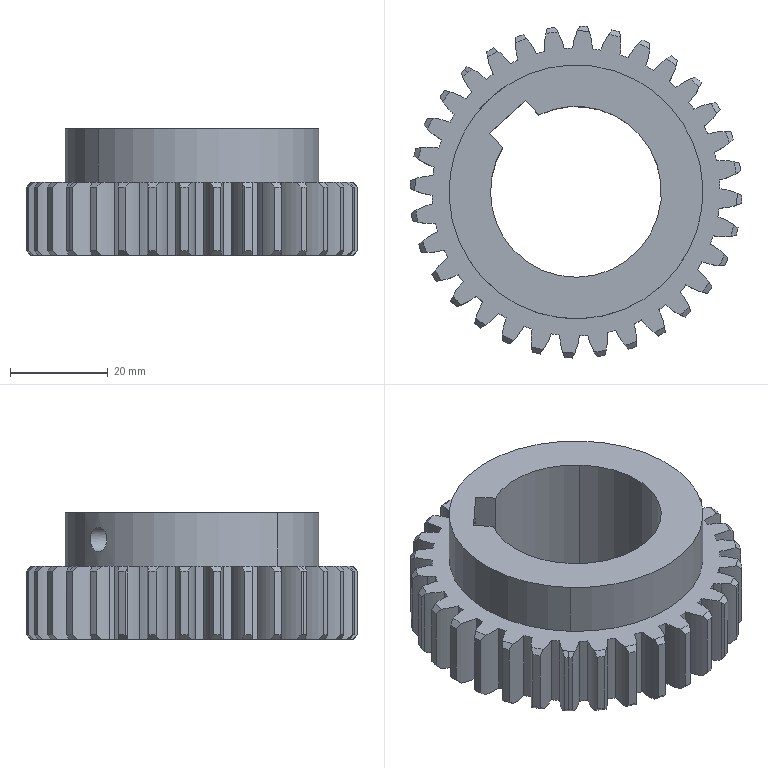Component | SolidWorks | Gear1-1 | 1 solid | 215 faces | volume 45009 mm3 | cylinder 140 | cone 69 | plane 6 | commonest cylinder face diameters 24.415 x68 68 x33 59 x32 35 x3 52 x2 5 x2